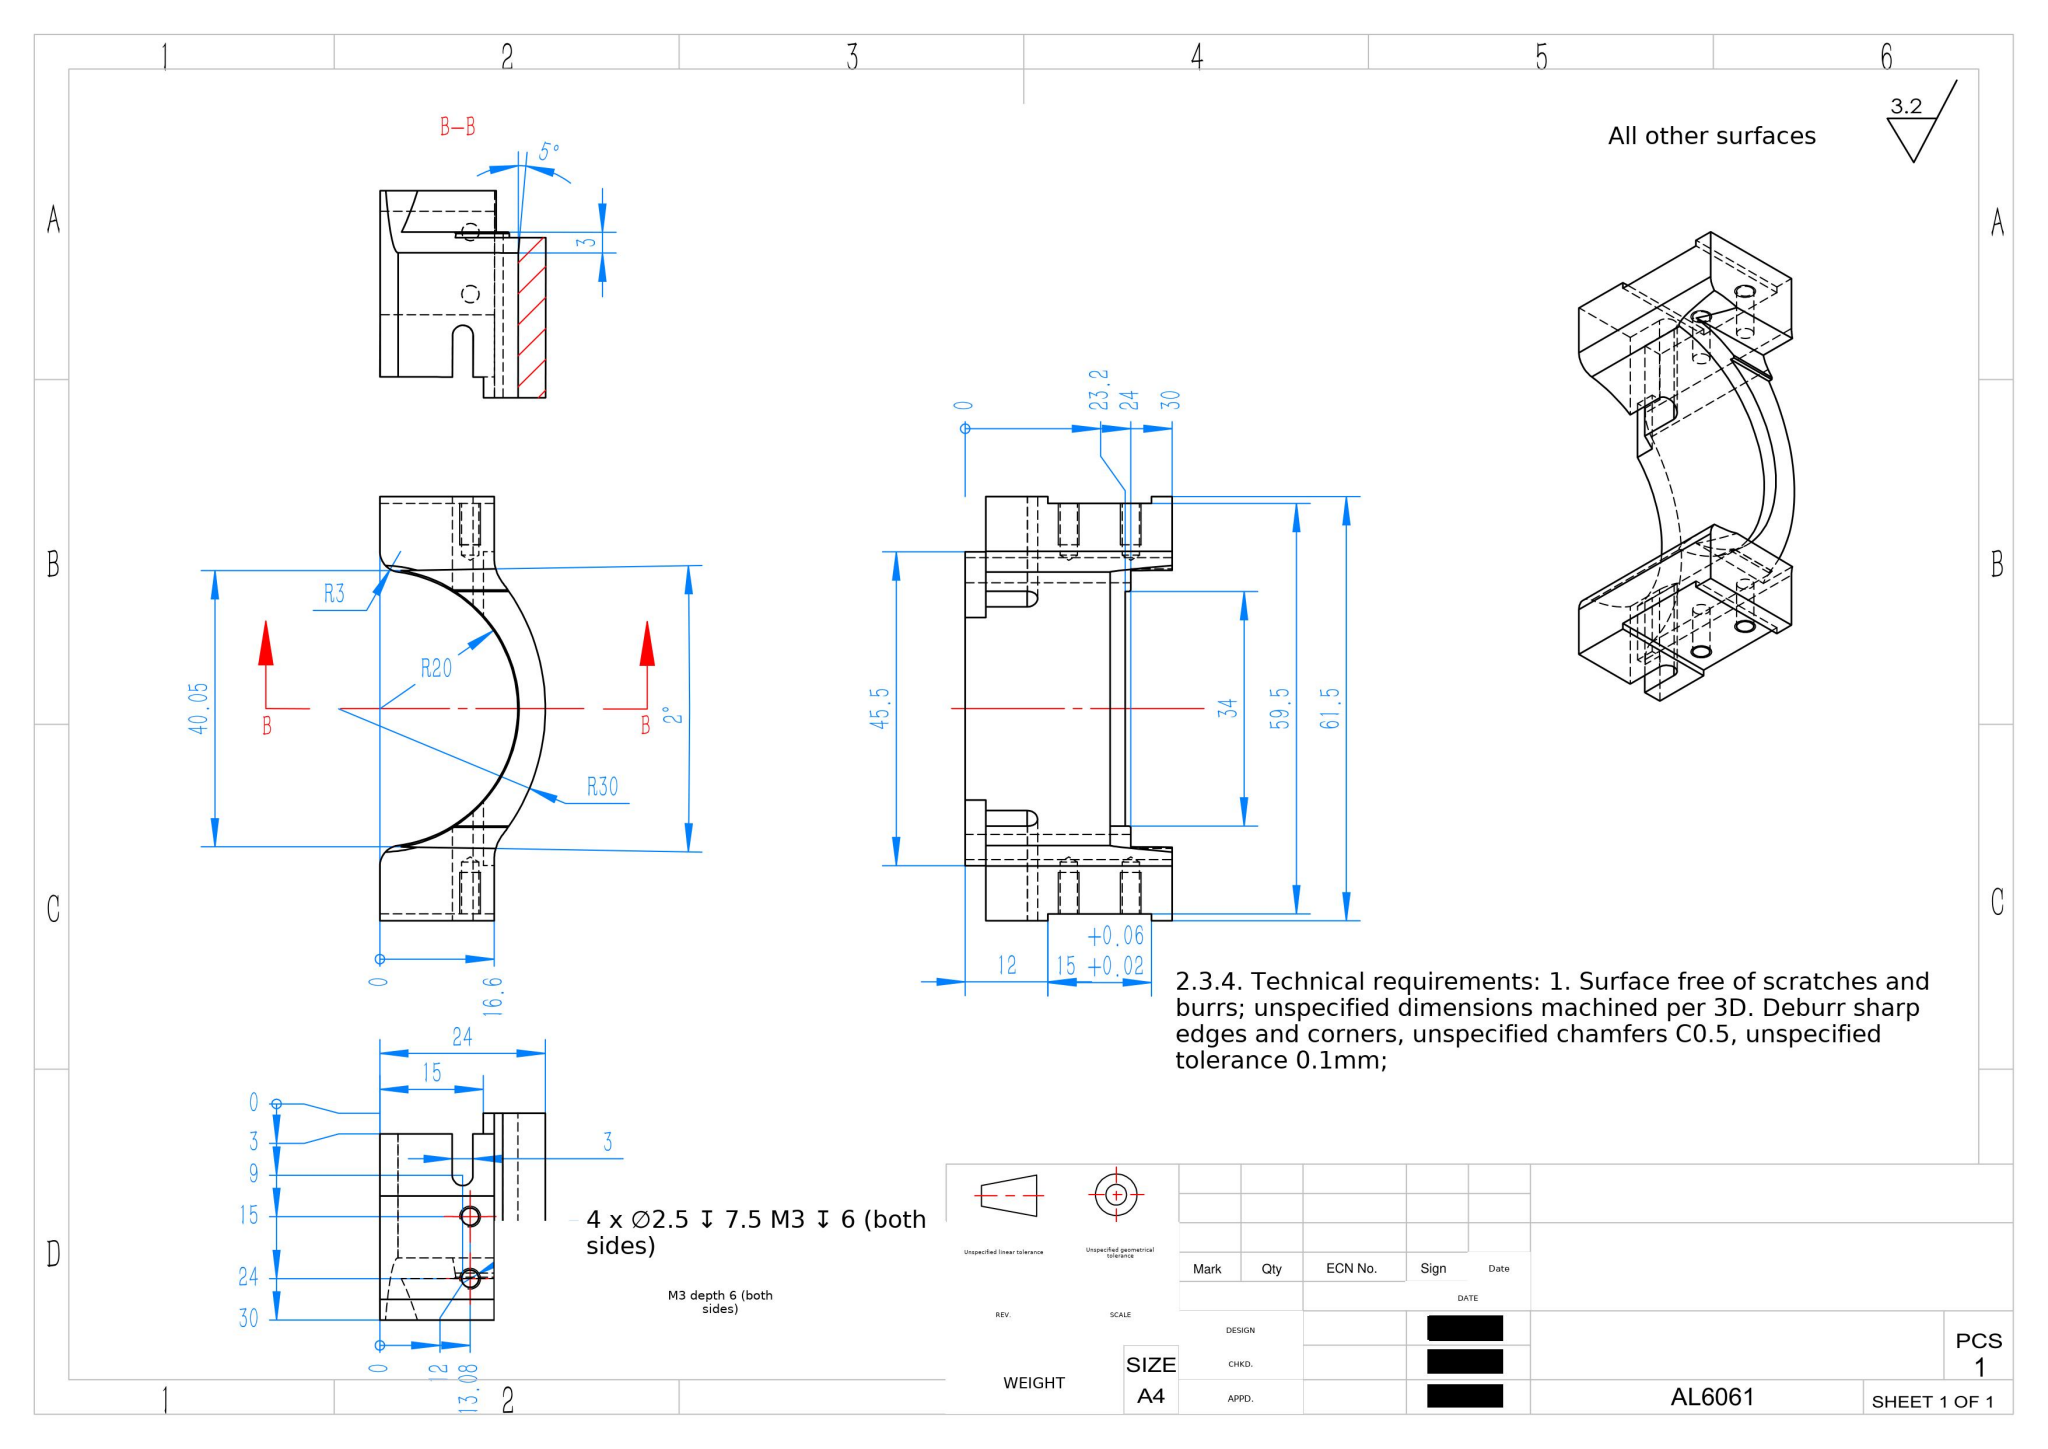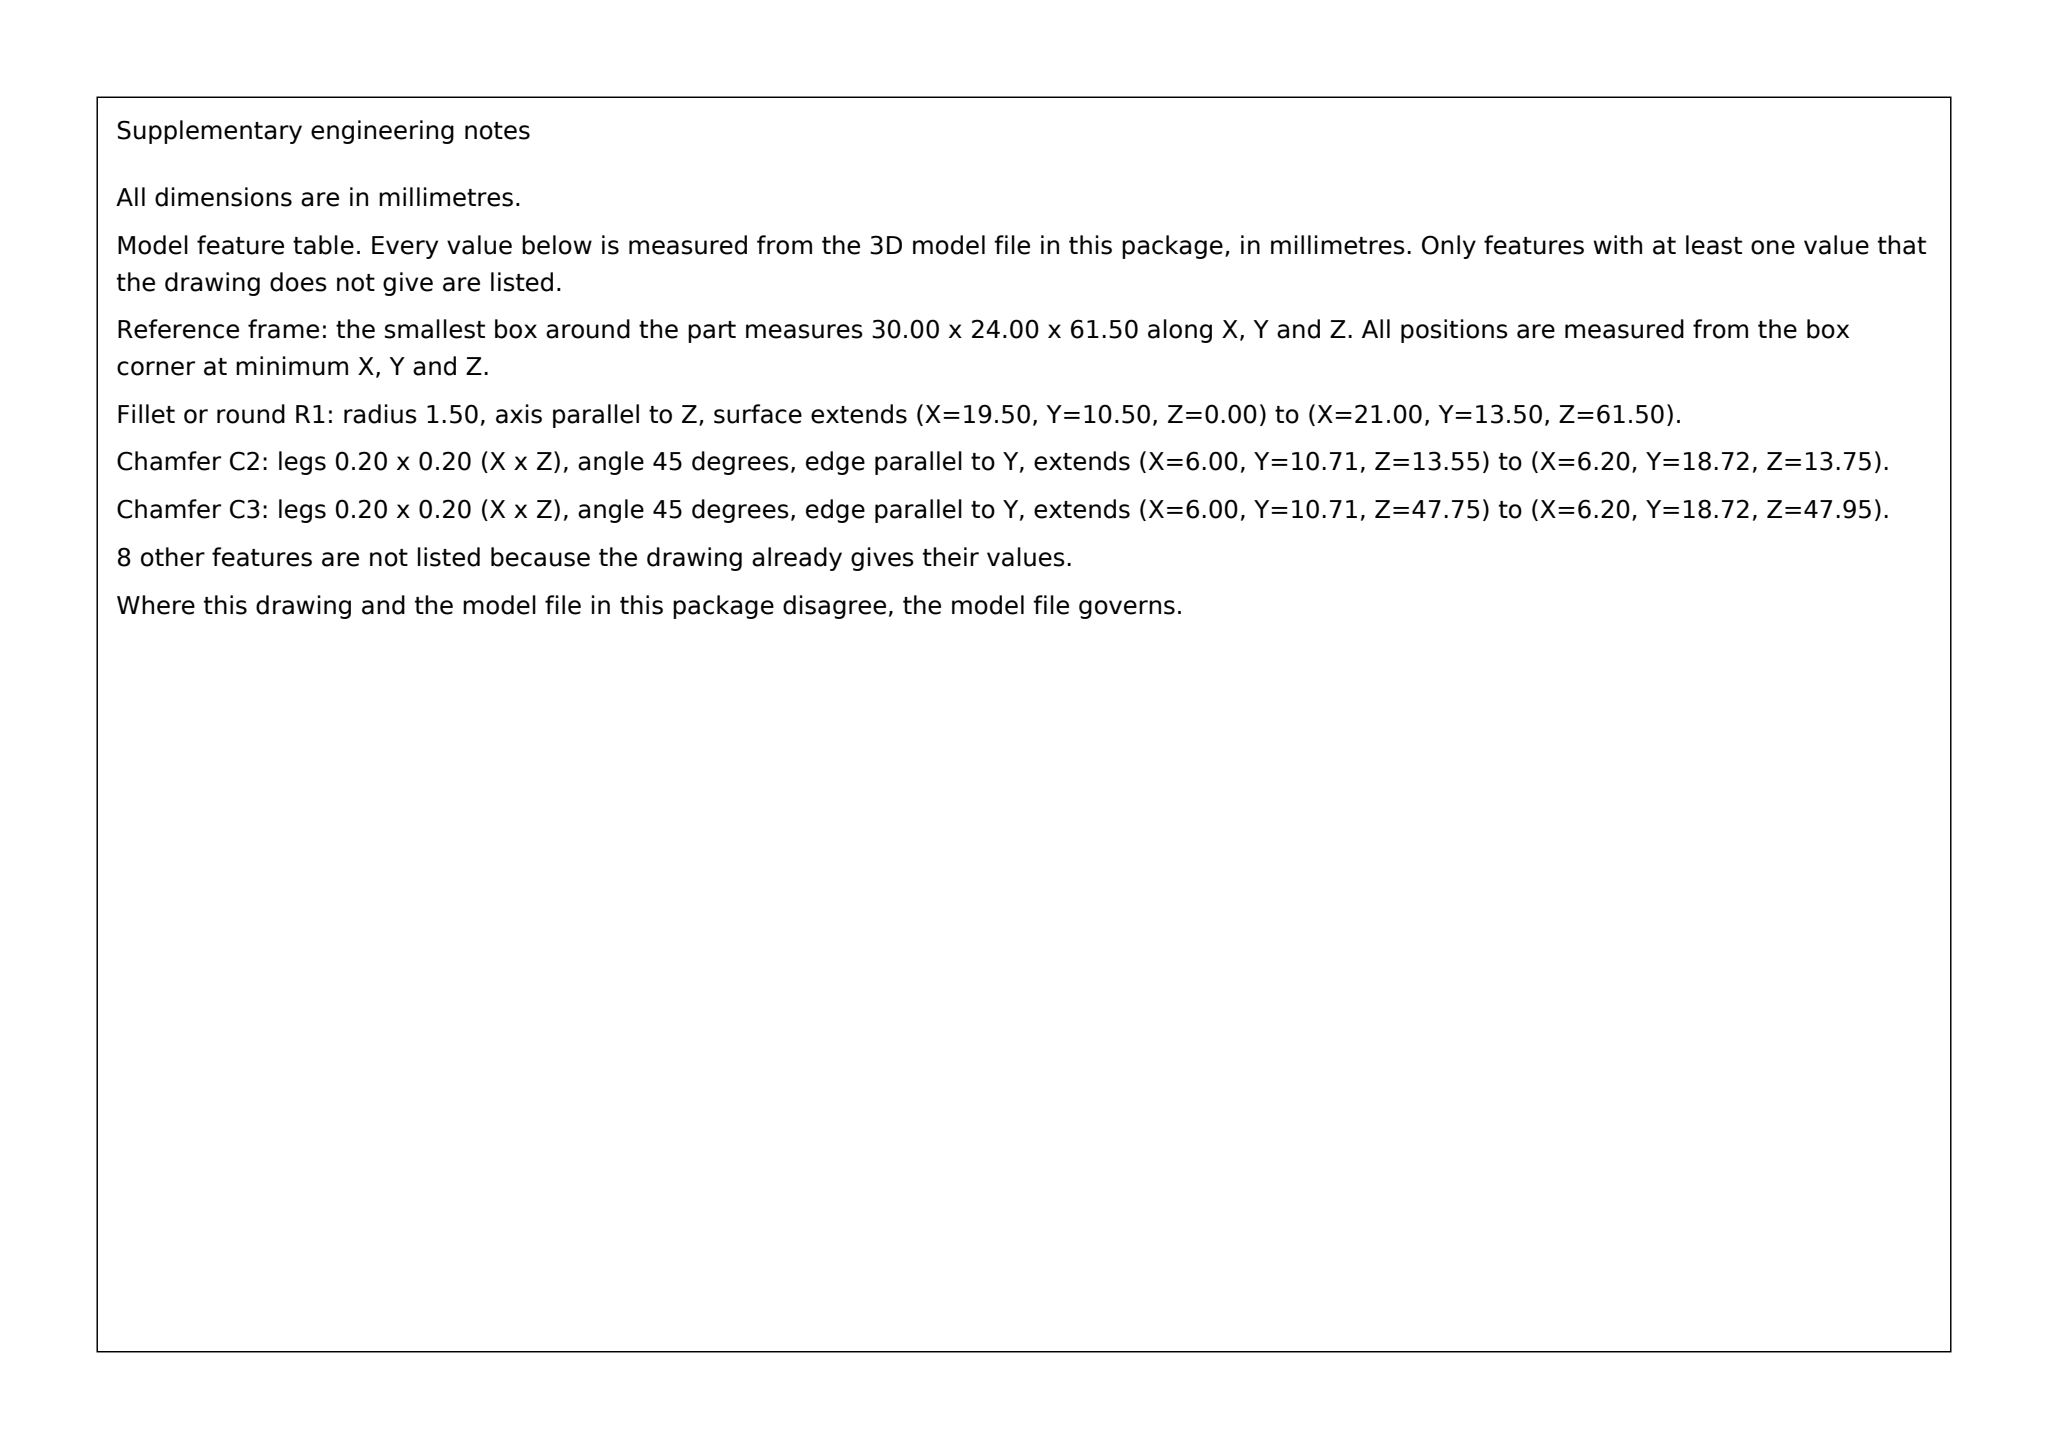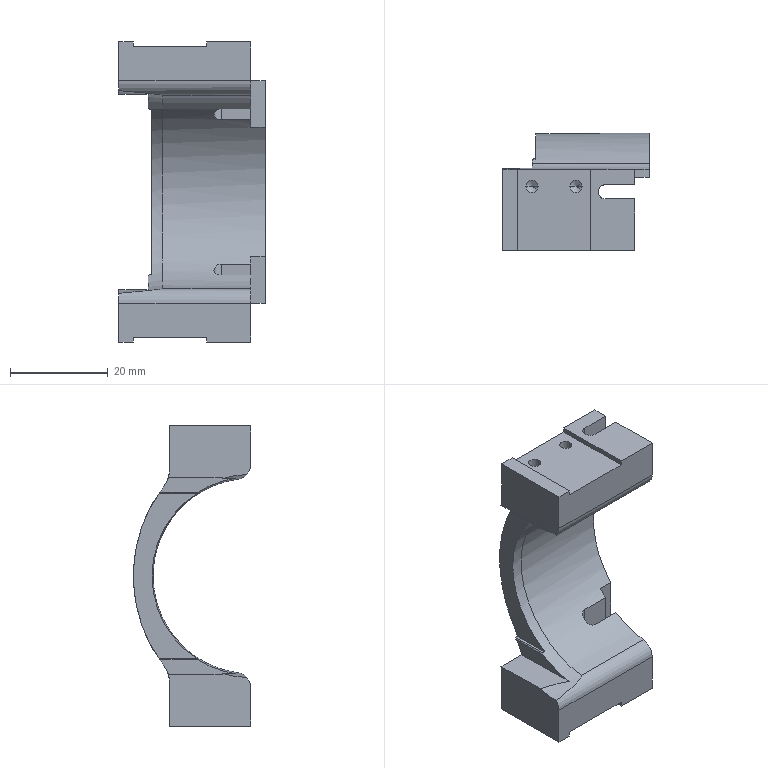Part | SolidWorks | mm | material AL6061 | 1 solid | 64 faces | box 30 x 24 x 61.5 mm | volume 13588 mm3 | plane 38 | cylinder 16 | cone 10 | commonest cylinder face diameters 2.5 x8 6 x2 12 x2 3 x2 40 x1 60 x1